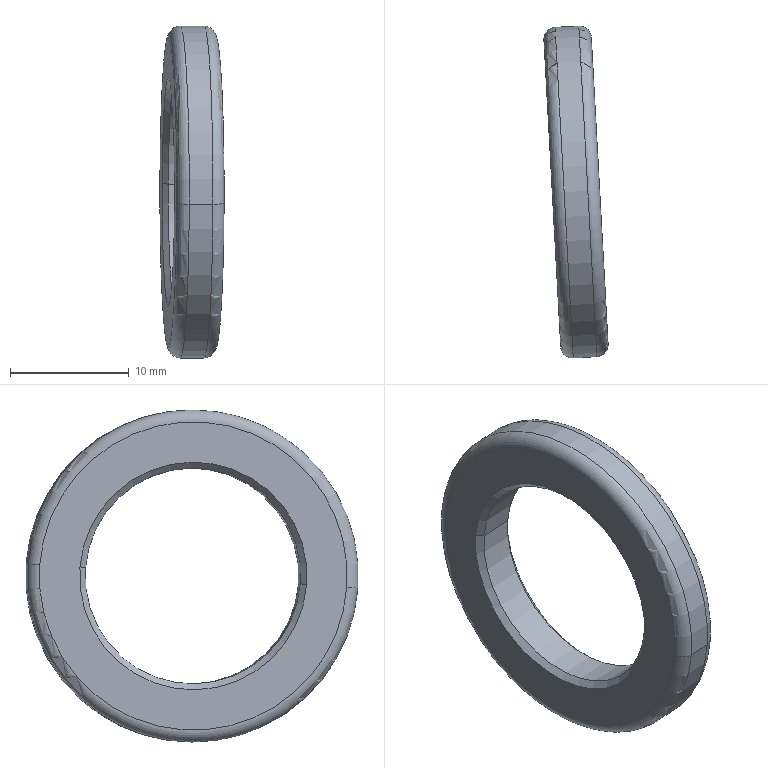Component | SolidWorks | T160418-M01U03-P10-1 | 1 solid | 14 faces | box 5.42 x 28.07 x 28 mm | volume 1371 mm3 | cone 4 | torus 4 | cylinder 4 | plane 2 | commonest cylinder face diameters 18.2 x2 28 x2 | material S45C
build123d program:
from build123d import *

# Parameters (mm, degrees)
SKETCH1_R           = 14
SKETCH1_R_2         = 9.1
BOSS_EXTRUDE1_DEPTH = 2
FILLET1_R           = 1
CHAMFER1_SIZE       = 0.5


with BuildPart() as part:
    # Sketch1 → Boss-Extrude1 (new, symmetric)
    with BuildSketch(Plane.XY):
        Circle(SKETCH1_R)
        Circle(SKETCH1_R_2, mode=Mode.SUBTRACT)
    extrude(amount=BOSS_EXTRUDE1_DEPTH, both=True)

    # Fillet1
    fillet1_edges = [part.edges().sort_by_distance(p)[0] for p in [
        (-14, 0, -2),
        (-14, 0, 2),
    ]]
    fillet(fillet1_edges, radius=FILLET1_R)

    # Chamfer1
    chamfer1_edges = [part.edges().sort_by_distance(p)[0] for p in [
        (-9.1, 0, -2),
        (-9.1, 0, 2),
    ]]
    chamfer(chamfer1_edges, length=CHAMFER1_SIZE)


solid = part.part

# Placed as in the assembly
solid = solid.moved(Location((495.31, 108.541, -217.818), (-90, 86.863, -74.264)))
STEP:
#1=COLOUR_RGB('',0.7922,0.8196,0.9333);
#2=FILL_AREA_STYLE_COLOUR('',#1);
#3=FILL_AREA_STYLE('',(#2));
#4=SURFACE_STYLE_FILL_AREA(#3);
#5=SURFACE_SIDE_STYLE('',(#4));
#6=SURFACE_STYLE_USAGE(.BOTH.,#5);
#7=PRESENTATION_STYLE_ASSIGNMENT((#6));
#8=CARTESIAN_POINT('',(19.461,3.913,-8.602));
#9=VERTEX_POINT('',#8);
#10=CARTESIAN_POINT('',(19.422,4.627,-8.549));
#11=VERTEX_POINT('',#10);
#12=CARTESIAN_POINT('',(19.441,4.27,-8.576));
#13=DIRECTION('',(-0.9985,-0.05472,-0.));
#14=DIRECTION('',(-0.05457,0.9958,0.07337));
#15=AXIS2_PLACEMENT_3D('',#12,#13,#14);
#16=CIRCLE('',#15,0.3583);
#17=EDGE_CURVE('',#9,#11,#16,.T.);
#18=ORIENTED_EDGE('',*,*,#17,.F.);
#19=CARTESIAN_POINT('',(19.442,3.893,-8.603));
#20=VERTEX_POINT('',#19);
#21=CARTESIAN_POINT('',(19.461,3.913,-8.602));
#22=DIRECTION('',(-0.6675,-0.7428,-0.05188));
#23=VECTOR('',#22,39.37);
#24=LINE('',#21,#23);
#25=EDGE_CURVE('',#9,#20,#24,.T.);
#26=ORIENTED_EDGE('',*,*,#25,.T.);
#27=CARTESIAN_POINT('',(19.401,4.645,-8.548));
#28=VERTEX_POINT('',#27);
#29=CARTESIAN_POINT('',(19.422,4.269,-8.576));
#30=DIRECTION('',(0.9985,0.05472,0.));
#31=DIRECTION('',(-0.05457,0.9958,0.07337));
#32=AXIS2_PLACEMENT_3D('',#29,#30,#31);
#33=CIRCLE('',#32,0.378);
#34=EDGE_CURVE('',#28,#20,#33,.T.);
#35=ORIENTED_EDGE('',*,*,#34,.F.);
#36=CARTESIAN_POINT('',(19.422,4.627,-8.549));
#37=DIRECTION('',(-0.7446,0.6655,0.05188));
#38=VECTOR('',#37,39.37);
#39=LINE('',#36,#38);
#40=EDGE_CURVE('',#11,#28,#39,.T.);
#41=ORIENTED_EDGE('',*,*,#40,.F.);
#42=EDGE_LOOP('',(#18,#26,#35,#41));
#43=FACE_OUTER_BOUND('',#42,.T.);
#44=CARTESIAN_POINT('',(19.441,4.27,-8.576));
#45=DIRECTION('',(-0.9985,-0.05472,-0.));
#46=DIRECTION('',(-0.05457,0.9958,0.07337));
#47=AXIS2_PLACEMENT_3D('',#44,#45,#46);
#48=CONICAL_SURFACE('',#47,0.3583,0.7854);
#49=ADVANCED_FACE('',(#43),#48,.F.);
#50=CARTESIAN_POINT('',(19.54,4.633,-8.549));
#51=VERTEX_POINT('',#50);
#52=CARTESIAN_POINT('',(19.579,3.92,-8.602));
#53=VERTEX_POINT('',#52);
#54=CARTESIAN_POINT('',(19.559,4.277,-8.576));
#55=DIRECTION('',(0.9985,0.05472,0.));
#56=DIRECTION('',(-0.05457,0.9958,0.07337));
#57=AXIS2_PLACEMENT_3D('',#54,#55,#56);
#58=CIRCLE('',#57,0.3583);
#59=EDGE_CURVE('',#51,#53,#58,.T.);
#60=ORIENTED_EDGE('',*,*,#59,.F.);
#61=CARTESIAN_POINT('',(19.558,4.654,-8.548));
#62=VERTEX_POINT('',#61);
#63=CARTESIAN_POINT('',(19.558,4.654,-8.548));
#64=DIRECTION('',(0.6675,0.7428,0.05188));
#65=VECTOR('',#64,39.37);
#66=LINE('',#63,#65);
#67=EDGE_CURVE('',#51,#62,#66,.T.);
#68=ORIENTED_EDGE('',*,*,#67,.T.);
#69=CARTESIAN_POINT('',(19.6,3.901,-8.603));
#70=VERTEX_POINT('',#69);
#71=CARTESIAN_POINT('',(19.579,4.278,-8.576));
#72=DIRECTION('',(-0.9985,-0.05472,-0.));
#73=DIRECTION('',(-0.05457,0.9958,0.07337));
#74=AXIS2_PLACEMENT_3D('',#71,#72,#73);
#75=CIRCLE('',#74,0.378);
#76=EDGE_CURVE('',#70,#62,#75,.T.);
#77=ORIENTED_EDGE('',*,*,#76,.F.);
#78=CARTESIAN_POINT('',(19.6,3.901,-8.603));
#79=DIRECTION('',(0.7446,-0.6655,-0.05188));
#80=VECTOR('',#79,39.37);
#81=LINE('',#78,#80);
#82=EDGE_CURVE('',#53,#70,#81,.T.);
#83=ORIENTED_EDGE('',*,*,#82,.F.);
#84=EDGE_LOOP('',(#60,#68,#77,#83));
#85=FACE_OUTER_BOUND('',#84,.T.);
#86=CARTESIAN_POINT('',(19.579,4.278,-8.576));
#87=DIRECTION('',(0.9985,0.05472,0.));
#88=DIRECTION('',(0.05457,-0.9958,-0.07337));
#89=AXIS2_PLACEMENT_3D('',#86,#87,#88);
#90=CONICAL_SURFACE('',#89,0.378,0.7854);
#91=ADVANCED_FACE('',(#85),#90,.F.);
#92=CARTESIAN_POINT('',(19.491,3.722,-8.616));
#93=VERTEX_POINT('',#92);
#94=CARTESIAN_POINT('',(19.431,4.82,-8.535));
#95=VERTEX_POINT('',#94);
#96=CARTESIAN_POINT('',(19.461,4.271,-8.576));
#97=DIRECTION('',(0.9985,0.05472,0.));
#98=DIRECTION('',(-0.05457,0.9958,0.07337));
#99=AXIS2_PLACEMENT_3D('',#96,#97,#98);
#100=CIRCLE('',#99,0.5512);
#101=EDGE_CURVE('',#93,#95,#100,.T.);
#102=ORIENTED_EDGE('',*,*,#101,.F.);
#103=CARTESIAN_POINT('',(19.45,3.759,-8.613));
#104=VERTEX_POINT('',#103);
#105=CARTESIAN_POINT('',(19.489,3.761,-8.613));
#106=DIRECTION('',(-0.004015,0.07326,-0.9973));
#107=DIRECTION('',(0.,0.9973,0.07326));
#108=AXIS2_PLACEMENT_3D('',#105,#106,#107);
#109=CIRCLE('',#108,0.03937);
#110=EDGE_CURVE('',#93,#104,#109,.T.);
#111=ORIENTED_EDGE('',*,*,#110,.T.);
#112=CARTESIAN_POINT('',(19.394,4.779,-8.538));
#113=VERTEX_POINT('',#112);
#114=CARTESIAN_POINT('',(19.422,4.269,-8.576));
#115=DIRECTION('',(-0.9985,-0.05472,-0.));
#116=DIRECTION('',(-0.05457,0.9958,0.07337));
#117=AXIS2_PLACEMENT_3D('',#114,#115,#116);
#118=CIRCLE('',#117,0.5118);
#119=EDGE_CURVE('',#113,#104,#118,.T.);
#120=ORIENTED_EDGE('',*,*,#119,.F.);
#121=CARTESIAN_POINT('',(19.433,4.781,-8.538));
#122=DIRECTION('',(0.004015,-0.07326,0.9973));
#123=DIRECTION('',(0.,-0.9973,-0.07326));
#124=AXIS2_PLACEMENT_3D('',#121,#122,#123);
#125=CIRCLE('',#124,0.03937);
#126=EDGE_CURVE('',#95,#113,#125,.T.);
#127=ORIENTED_EDGE('',*,*,#126,.F.);
#128=EDGE_LOOP('',(#102,#111,#120,#127));
#129=FACE_OUTER_BOUND('',#128,.T.);
#130=CARTESIAN_POINT('',(19.461,4.271,-8.576));
#131=DIRECTION('',(-0.9985,-0.05472,-0.));
#132=DIRECTION('',(-0.05457,0.9958,0.07337));
#133=AXIS2_PLACEMENT_3D('',#130,#131,#132);
#134=TOROIDAL_SURFACE('',#133,0.5118,0.03937);
#135=ADVANCED_FACE('',(#129),#134,.T.);
#136=CARTESIAN_POINT('',(19.607,3.768,-8.613));
#137=VERTEX_POINT('',#136);
#138=CARTESIAN_POINT('',(19.551,4.787,-8.538));
#139=VERTEX_POINT('',#138);
#140=CARTESIAN_POINT('',(19.579,4.278,-8.576));
#141=DIRECTION('',(0.9985,0.05472,0.));
#142=DIRECTION('',(-0.05457,0.9958,0.07337));
#143=AXIS2_PLACEMENT_3D('',#140,#141,#142);
#144=CIRCLE('',#143,0.5118);
#145=EDGE_CURVE('',#137,#139,#144,.T.);
#146=ORIENTED_EDGE('',*,*,#145,.F.);
#147=CARTESIAN_POINT('',(19.57,3.727,-8.616));
#148=VERTEX_POINT('',#147);
#149=CARTESIAN_POINT('',(19.568,3.766,-8.613));
#150=DIRECTION('',(-0.004015,0.07326,-0.9973));
#151=DIRECTION('',(0.,0.9973,0.07326));
#152=AXIS2_PLACEMENT_3D('',#149,#150,#151);
#153=CIRCLE('',#152,0.03937);
#154=EDGE_CURVE('',#137,#148,#153,.T.);
#155=ORIENTED_EDGE('',*,*,#154,.T.);
#156=CARTESIAN_POINT('',(19.51,4.824,-8.535));
#157=VERTEX_POINT('',#156);
#158=CARTESIAN_POINT('',(19.54,4.275,-8.576));
#159=DIRECTION('',(-0.9985,-0.05472,-0.));
#160=DIRECTION('',(-0.05457,0.9958,0.07337));
#161=AXIS2_PLACEMENT_3D('',#158,#159,#160);
#162=CIRCLE('',#161,0.5512);
#163=EDGE_CURVE('',#157,#148,#162,.T.);
#164=ORIENTED_EDGE('',*,*,#163,.F.);
#165=CARTESIAN_POINT('',(19.512,4.785,-8.538));
#166=DIRECTION('',(0.004015,-0.07326,0.9973));
#167=DIRECTION('',(0.,-0.9973,-0.07326));
#168=AXIS2_PLACEMENT_3D('',#165,#166,#167);
#169=CIRCLE('',#168,0.03937);
#170=EDGE_CURVE('',#139,#157,#169,.T.);
#171=ORIENTED_EDGE('',*,*,#170,.F.);
#172=EDGE_LOOP('',(#146,#155,#164,#171));
#173=FACE_OUTER_BOUND('',#172,.T.);
#174=CARTESIAN_POINT('',(19.54,4.275,-8.576));
#175=DIRECTION('',(-0.9985,-0.05472,-0.));
#176=DIRECTION('',(-0.05457,0.9958,0.07337));
#177=AXIS2_PLACEMENT_3D('',#174,#175,#176);
#178=TOROIDAL_SURFACE('',#177,0.5118,0.03937);
#179=ADVANCED_FACE('',(#173),#178,.T.);
#180=ORIENTED_EDGE('',*,*,#17,.T.);
#181=CARTESIAN_POINT('',(19.402,4.626,-8.549));
#182=DIRECTION('',(0.9985,0.05472,0.));
#183=VECTOR('',#182,39.37);
#184=LINE('',#181,#183);
#185=EDGE_CURVE('',#11,#51,#184,.T.);
#186=ORIENTED_EDGE('',*,*,#185,.T.);
#187=ORIENTED_EDGE('',*,*,#59,.T.);
#188=CARTESIAN_POINT('',(19.441,3.912,-8.602));
#189=DIRECTION('',(0.9985,0.05472,0.));
#190=VECTOR('',#189,39.37);
#191=LINE('',#188,#190);
#192=EDGE_CURVE('',#9,#53,#191,.T.);
#193=ORIENTED_EDGE('',*,*,#192,.F.);
#194=EDGE_LOOP('',(#180,#186,#187,#193));
#195=FACE_OUTER_BOUND('',#194,.T.);
#196=CARTESIAN_POINT('',(19.422,4.269,-8.576));
#197=DIRECTION('',(0.9985,0.05472,0.));
#198=DIRECTION('',(0.05457,-0.9958,-0.07337));
#199=AXIS2_PLACEMENT_3D('',#196,#197,#198);
#200=CYLINDRICAL_SURFACE('',#199,0.3583);
#201=ADVANCED_FACE('',(#195),#200,.F.);
#202=ORIENTED_EDGE('',*,*,#101,.T.);
#203=CARTESIAN_POINT('',(19.392,4.818,-8.535));
#204=DIRECTION('',(0.9985,0.05472,0.));
#205=VECTOR('',#204,39.37);
#206=LINE('',#203,#205);
#207=EDGE_CURVE('',#95,#157,#206,.T.);
#208=ORIENTED_EDGE('',*,*,#207,.T.);
#209=ORIENTED_EDGE('',*,*,#163,.T.);
#210=CARTESIAN_POINT('',(19.452,3.72,-8.616));
#211=DIRECTION('',(0.9985,0.05472,0.));
#212=VECTOR('',#211,39.37);
#213=LINE('',#210,#212);
#214=EDGE_CURVE('',#93,#148,#213,.T.);
#215=ORIENTED_EDGE('',*,*,#214,.F.);
#216=EDGE_LOOP('',(#202,#208,#209,#215));
#217=FACE_OUTER_BOUND('',#216,.T.);
#218=CARTESIAN_POINT('',(19.422,4.269,-8.576));
#219=DIRECTION('',(0.9985,0.05472,0.));
#220=DIRECTION('',(0.05457,-0.9958,-0.07337));
#221=AXIS2_PLACEMENT_3D('',#218,#219,#220);
#222=CYLINDRICAL_SURFACE('',#221,0.5512);
#223=ADVANCED_FACE('',(#217),#222,.T.);
#224=ORIENTED_EDGE('',*,*,#34,.T.);
#225=CARTESIAN_POINT('',(19.422,4.269,-8.576));
#226=DIRECTION('',(0.9985,0.05472,0.));
#227=DIRECTION('',(-0.05457,0.9958,0.07337));
#228=AXIS2_PLACEMENT_3D('',#225,#226,#227);
#229=CIRCLE('',#228,0.378);
#230=EDGE_CURVE('',#20,#28,#229,.T.);
#231=ORIENTED_EDGE('',*,*,#230,.T.);
#232=EDGE_LOOP('',(#224,#231));
#233=FACE_BOUND('',#232,.T.);
#234=ORIENTED_EDGE('',*,*,#119,.T.);
#235=CARTESIAN_POINT('',(19.422,4.269,-8.576));
#236=DIRECTION('',(-0.9985,-0.05472,-0.));
#237=DIRECTION('',(-0.05457,0.9958,0.07337));
#238=AXIS2_PLACEMENT_3D('',#235,#236,#237);
#239=CIRCLE('',#238,0.5118);
#240=EDGE_CURVE('',#104,#113,#239,.T.);
#241=ORIENTED_EDGE('',*,*,#240,.T.);
#242=EDGE_LOOP('',(#234,#241));
#243=FACE_OUTER_BOUND('',#242,.T.);
#244=CARTESIAN_POINT('',(19.422,4.269,-8.576));
#245=DIRECTION('',(-0.9985,-0.05472,-0.));
#246=DIRECTION('',(-0.05457,0.9958,0.07337));
#247=AXIS2_PLACEMENT_3D('',#244,#245,#246);
#248=PLANE('',#247);
#249=ADVANCED_FACE('',(#233,#243),#248,.T.);
#250=ORIENTED_EDGE('',*,*,#76,.T.);
#251=CARTESIAN_POINT('',(19.579,4.278,-8.576));
#252=DIRECTION('',(-0.9985,-0.05472,-0.));
#253=DIRECTION('',(-0.05457,0.9958,0.07337));
#254=AXIS2_PLACEMENT_3D('',#251,#252,#253);
#255=CIRCLE('',#254,0.378);
#256=EDGE_CURVE('',#62,#70,#255,.T.);
#257=ORIENTED_EDGE('',*,*,#256,.T.);
#258=EDGE_LOOP('',(#250,#257));
#259=FACE_BOUND('',#258,.T.);
#260=CARTESIAN_POINT('',(19.579,4.278,-8.576));
#261=DIRECTION('',(0.9985,0.05472,0.));
#262=DIRECTION('',(-0.05457,0.9958,0.07337));
#263=AXIS2_PLACEMENT_3D('',#260,#261,#262);
#264=CIRCLE('',#263,0.5118);
#265=EDGE_CURVE('',#139,#137,#264,.T.);
#266=ORIENTED_EDGE('',*,*,#265,.T.);
#267=ORIENTED_EDGE('',*,*,#145,.T.);
#268=EDGE_LOOP('',(#266,#267));
#269=FACE_OUTER_BOUND('',#268,.T.);
#270=CARTESIAN_POINT('',(19.579,4.278,-8.576));
#271=DIRECTION('',(-0.9985,-0.05472,-0.));
#272=DIRECTION('',(-0.05457,0.9958,0.07337));
#273=AXIS2_PLACEMENT_3D('',#270,#271,#272);
#274=PLANE('',#273);
#275=ADVANCED_FACE('',(#259,#269),#274,.F.);
#276=ORIENTED_EDGE('',*,*,#207,.F.);
#277=CARTESIAN_POINT('',(19.461,4.271,-8.576));
#278=DIRECTION('',(0.9985,0.05472,0.));
#279=DIRECTION('',(-0.05457,0.9958,0.07337));
#280=AXIS2_PLACEMENT_3D('',#277,#278,#279);
#281=CIRCLE('',#280,0.5512);
#282=EDGE_CURVE('',#95,#93,#281,.T.);
#283=ORIENTED_EDGE('',*,*,#282,.T.);
#284=ORIENTED_EDGE('',*,*,#214,.T.);
#285=CARTESIAN_POINT('',(19.54,4.275,-8.576));
#286=DIRECTION('',(-0.9985,-0.05472,-0.));
#287=DIRECTION('',(-0.05457,0.9958,0.07337));
#288=AXIS2_PLACEMENT_3D('',#285,#286,#287);
#289=CIRCLE('',#288,0.5512);
#290=EDGE_CURVE('',#148,#157,#289,.T.);
#291=ORIENTED_EDGE('',*,*,#290,.T.);
#292=EDGE_LOOP('',(#276,#283,#284,#291));
#293=FACE_OUTER_BOUND('',#292,.T.);
#294=CARTESIAN_POINT('',(19.422,4.269,-8.576));
#295=DIRECTION('',(0.9985,0.05472,0.));
#296=DIRECTION('',(0.05457,-0.9958,-0.07337));
#297=AXIS2_PLACEMENT_3D('',#294,#295,#296);
#298=CYLINDRICAL_SURFACE('',#297,0.5512);
#299=ADVANCED_FACE('',(#293),#298,.T.);
#300=ORIENTED_EDGE('',*,*,#185,.F.);
#301=CARTESIAN_POINT('',(19.441,4.27,-8.576));
#302=DIRECTION('',(-0.9985,-0.05472,-0.));
#303=DIRECTION('',(-0.05457,0.9958,0.07337));
#304=AXIS2_PLACEMENT_3D('',#301,#302,#303);
#305=CIRCLE('',#304,0.3583);
#306=EDGE_CURVE('',#11,#9,#305,.T.);
#307=ORIENTED_EDGE('',*,*,#306,.T.);
#308=ORIENTED_EDGE('',*,*,#192,.T.);
#309=CARTESIAN_POINT('',(19.559,4.277,-8.576));
#310=DIRECTION('',(0.9985,0.05472,0.));
#311=DIRECTION('',(-0.05457,0.9958,0.07337));
#312=AXIS2_PLACEMENT_3D('',#309,#310,#311);
#313=CIRCLE('',#312,0.3583);
#314=EDGE_CURVE('',#53,#51,#313,.T.);
#315=ORIENTED_EDGE('',*,*,#314,.T.);
#316=EDGE_LOOP('',(#300,#307,#308,#315));
#317=FACE_OUTER_BOUND('',#316,.T.);
#318=CARTESIAN_POINT('',(19.422,4.269,-8.576));
#319=DIRECTION('',(0.9985,0.05472,0.));
#320=DIRECTION('',(0.05457,-0.9958,-0.07337));
#321=AXIS2_PLACEMENT_3D('',#318,#319,#320);
#322=CYLINDRICAL_SURFACE('',#321,0.3583);
#323=ADVANCED_FACE('',(#317),#322,.F.);
#324=ORIENTED_EDGE('',*,*,#154,.F.);
#325=ORIENTED_EDGE('',*,*,#265,.F.);
#326=ORIENTED_EDGE('',*,*,#170,.T.);
#327=ORIENTED_EDGE('',*,*,#290,.F.);
#328=EDGE_LOOP('',(#324,#325,#326,#327));
#329=FACE_OUTER_BOUND('',#328,.T.);
#330=CARTESIAN_POINT('',(19.54,4.275,-8.576));
#331=DIRECTION('',(-0.9985,-0.05472,-0.));
#332=DIRECTION('',(-0.05457,0.9958,0.07337));
#333=AXIS2_PLACEMENT_3D('',#330,#331,#332);
#334=TOROIDAL_SURFACE('',#333,0.5118,0.03937);
#335=ADVANCED_FACE('',(#329),#334,.T.);
#336=ORIENTED_EDGE('',*,*,#110,.F.);
#337=ORIENTED_EDGE('',*,*,#282,.F.);
#338=ORIENTED_EDGE('',*,*,#126,.T.);
#339=ORIENTED_EDGE('',*,*,#240,.F.);
#340=EDGE_LOOP('',(#336,#337,#338,#339));
#341=FACE_OUTER_BOUND('',#340,.T.);
#342=CARTESIAN_POINT('',(19.461,4.271,-8.576));
#343=DIRECTION('',(-0.9985,-0.05472,-0.));
#344=DIRECTION('',(-0.05457,0.9958,0.07337));
#345=AXIS2_PLACEMENT_3D('',#342,#343,#344);
#346=TOROIDAL_SURFACE('',#345,0.5118,0.03937);
#347=ADVANCED_FACE('',(#341),#346,.T.);
#348=ORIENTED_EDGE('',*,*,#67,.F.);
#349=ORIENTED_EDGE('',*,*,#314,.F.);
#350=ORIENTED_EDGE('',*,*,#82,.T.);
#351=ORIENTED_EDGE('',*,*,#256,.F.);
#352=EDGE_LOOP('',(#348,#349,#350,#351));
#353=FACE_OUTER_BOUND('',#352,.T.);
#354=CARTESIAN_POINT('',(19.579,4.278,-8.576));
#355=DIRECTION('',(0.9985,0.05472,0.));
#356=DIRECTION('',(0.05457,-0.9958,-0.07337));
#357=AXIS2_PLACEMENT_3D('',#354,#355,#356);
#358=CONICAL_SURFACE('',#357,0.378,0.7854);
#359=ADVANCED_FACE('',(#353),#358,.F.);
#360=ORIENTED_EDGE('',*,*,#25,.F.);
#361=ORIENTED_EDGE('',*,*,#306,.F.);
#362=ORIENTED_EDGE('',*,*,#40,.T.);
#363=ORIENTED_EDGE('',*,*,#230,.F.);
#364=EDGE_LOOP('',(#360,#361,#362,#363));
#365=FACE_OUTER_BOUND('',#364,.T.);
#366=CARTESIAN_POINT('',(19.441,4.27,-8.576));
#367=DIRECTION('',(-0.9985,-0.05472,-0.));
#368=DIRECTION('',(-0.05457,0.9958,0.07337));
#369=AXIS2_PLACEMENT_3D('',#366,#367,#368);
#370=CONICAL_SURFACE('',#369,0.3583,0.7854);
#371=ADVANCED_FACE('',(#365),#370,.F.);
#372=CLOSED_SHELL('',(#49,#91,#135,#179,#201,#223,#249,#275,#299,#323,#335,#347,#359,#371));
#373=MANIFOLD_SOLID_BREP('',#372);
#374=STYLED_ITEM('',(#7),#373);
#375=(LENGTH_UNIT()NAMED_UNIT(*)SI_UNIT($,.METRE.));
#376=LENGTH_MEASURE_WITH_UNIT(LENGTH_MEASURE(0.0254),#375);
#377=DIMENSIONAL_EXPONENTS(1.,0.,0.,0.,0.,0.,0.);
#378=(CONVERSION_BASED_UNIT('',#376)LENGTH_UNIT()NAMED_UNIT(#377));
#379=UNCERTAINTY_MEASURE_WITH_UNIT(LENGTH_MEASURE(0.00001),#378,'','');
#380=(NAMED_UNIT(*)PLANE_ANGLE_UNIT()SI_UNIT($,.RADIAN.));
#381=(NAMED_UNIT(*)SI_UNIT($,.STERADIAN.)SOLID_ANGLE_UNIT());
#382=(GEOMETRIC_REPRESENTATION_CONTEXT(3)GLOBAL_UNCERTAINTY_ASSIGNED_CONTEXT((#379))GLOBAL_UNIT_ASSIGNED_CONTEXT((#378,#380,#381))REPRESENTATION_CONTEXT('',''));
#383=MECHANICAL_DESIGN_GEOMETRIC_PRESENTATION_REPRESENTATION('',(#374),#382);
#384=PRESENTATION_LAYER_ASSIGNMENT('','',(#374));
#385=CARTESIAN_POINT('',(0.,0.,0.));
#386=DIRECTION('',(0.,0.,1.));
#387=DIRECTION('',(1.,0.,0.));
#388=AXIS2_PLACEMENT_3D('',#385,#386,#387);
#389=(LENGTH_UNIT()NAMED_UNIT(*)SI_UNIT($,.METRE.));
#390=LENGTH_MEASURE_WITH_UNIT(LENGTH_MEASURE(0.0254),#389);
#391=DIMENSIONAL_EXPONENTS(1.,0.,0.,0.,0.,0.,0.);
#392=(CONVERSION_BASED_UNIT('',#390)LENGTH_UNIT()NAMED_UNIT(#391));
#393=UNCERTAINTY_MEASURE_WITH_UNIT(LENGTH_MEASURE(0.00001),#392,'','');
#394=(NAMED_UNIT(*)PLANE_ANGLE_UNIT()SI_UNIT($,.RADIAN.));
#395=(NAMED_UNIT(*)SI_UNIT($,.STERADIAN.)SOLID_ANGLE_UNIT());
#396=(GEOMETRIC_REPRESENTATION_CONTEXT(3)GLOBAL_UNCERTAINTY_ASSIGNED_CONTEXT((#393))GLOBAL_UNIT_ASSIGNED_CONTEXT((#392,#394,#395))REPRESENTATION_CONTEXT('',''));
#397=ADVANCED_BREP_SHAPE_REPRESENTATION('',(#373,#388),#396);